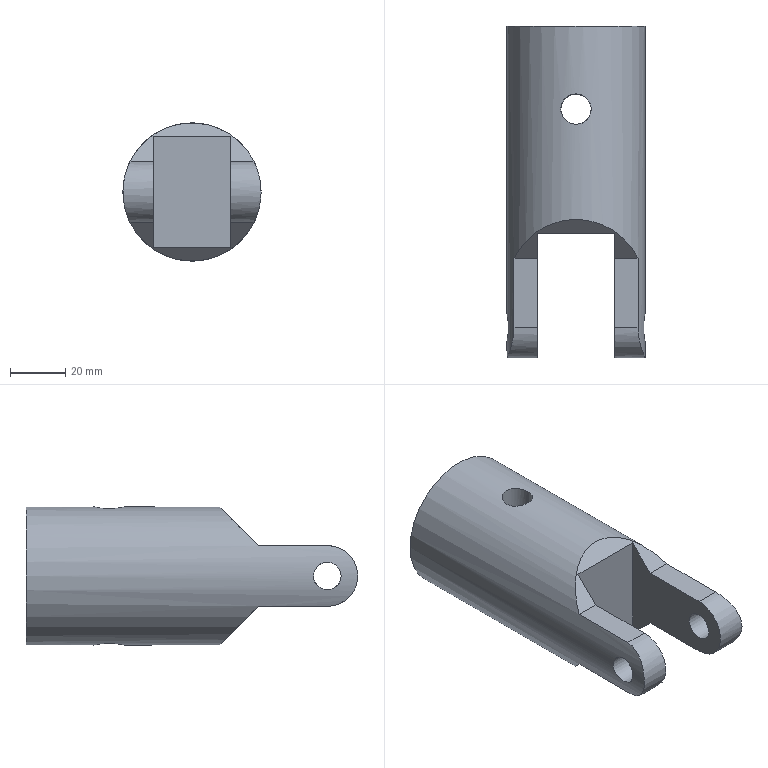Component | NX | UNIVERSAL_JOINT_CONNECTOR_MODEL1 | 1 solid | 19 faces | volume 125969 mm3 | plane 10 | cylinder 8 | cone 1 | commonest cylinder face diameters 22 x2 10 x2 11 x2 50 x1 30 x1